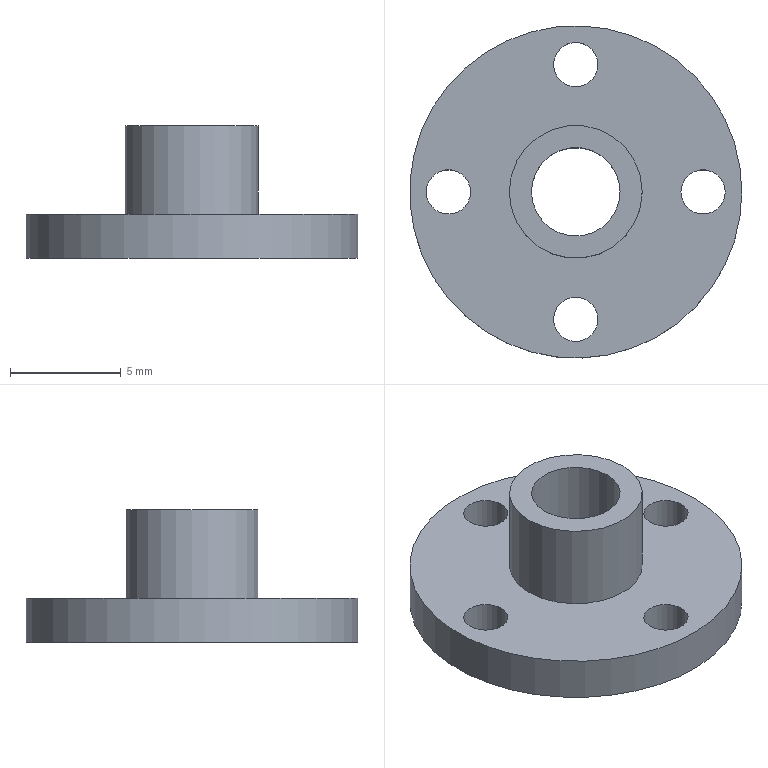Component | NX | EXT_PIPE_UPPER_END_COVER | 1 solid | 10 faces | volume 366 mm3 | cylinder 7 | plane 3 | commonest cylinder face diameters 2 x4 15 x1 6 x1 4 x1